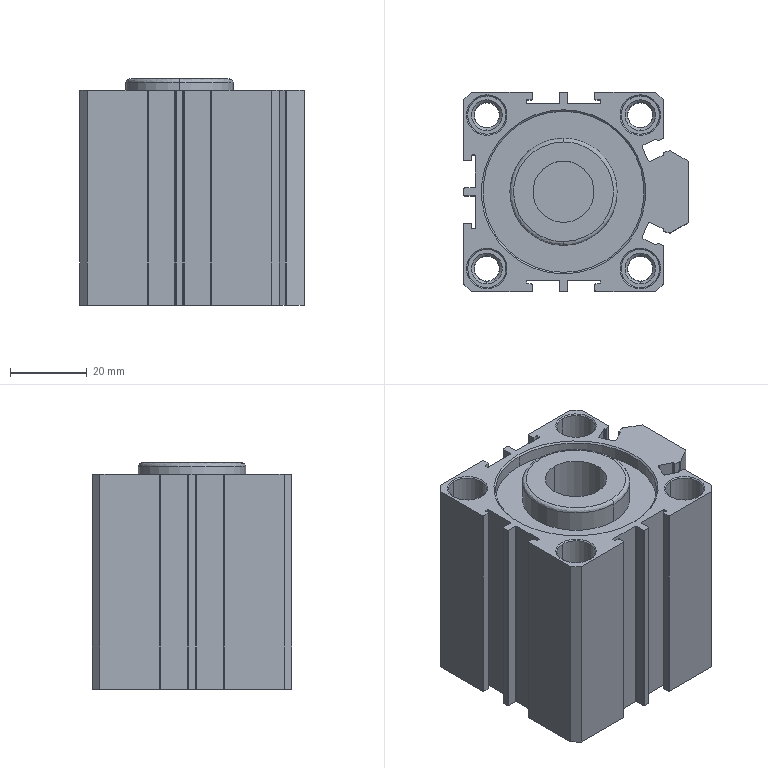Component | SolidWorks | SDA40x20SB_0_+_-1-1_SDAS-40x2020_b-1-dx-1 | 1 solid | 255 faces | volume 79851 mm3 | cylinder 110 | plane 87 | cone 56 | spline 2 | commonest cylinder face diameters 0.4 x46 10 x16 6.647 x16 0.8 x10 6.5 x8 40 x4 8.566 x4 16 x2